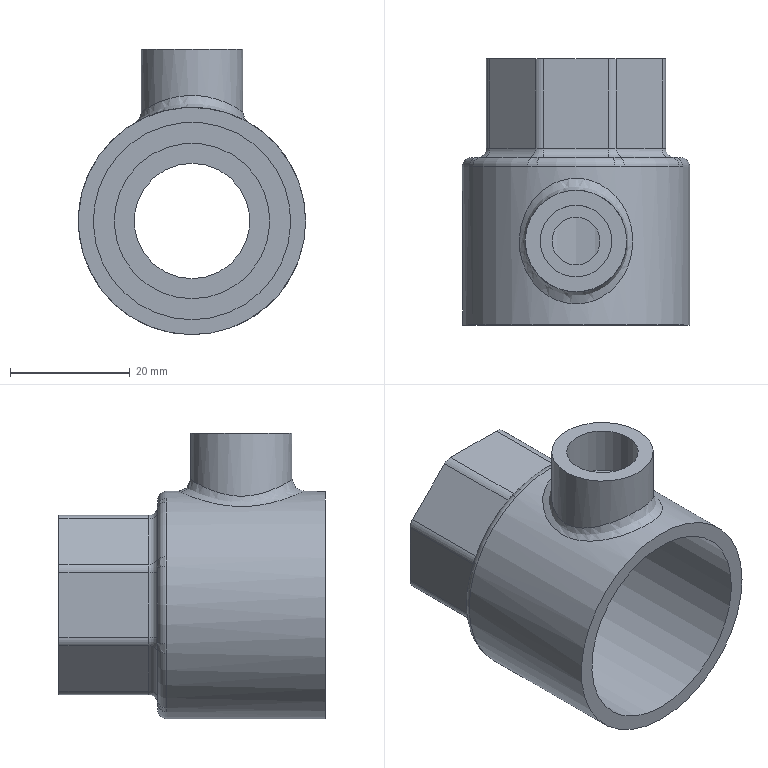Component | NX | VALVE_BODY | 1 solid | 74 faces | volume 15284 mm3 | cylinder 25 | plane 24 | torus 16 | spline 9 | commonest cylinder face diameters 4 x8 3 x8 38 x1 17 x1 33 x1 26 x1 19.304 x1 25.146 x1